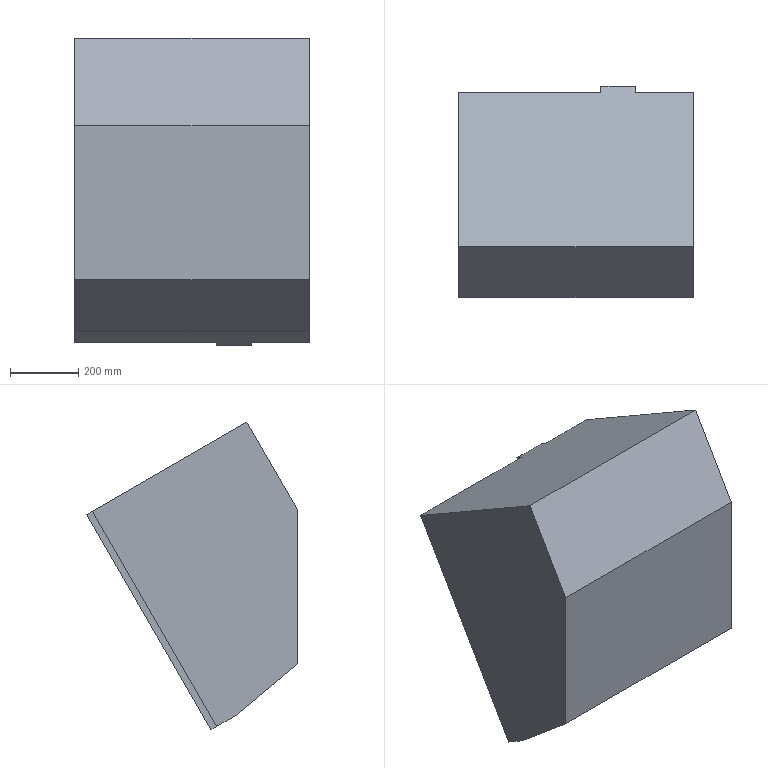Component | NX | SIM15_X2_SCHLITTEN | 1 solid | 12 faces | volume 222056121 mm3 | plane 12